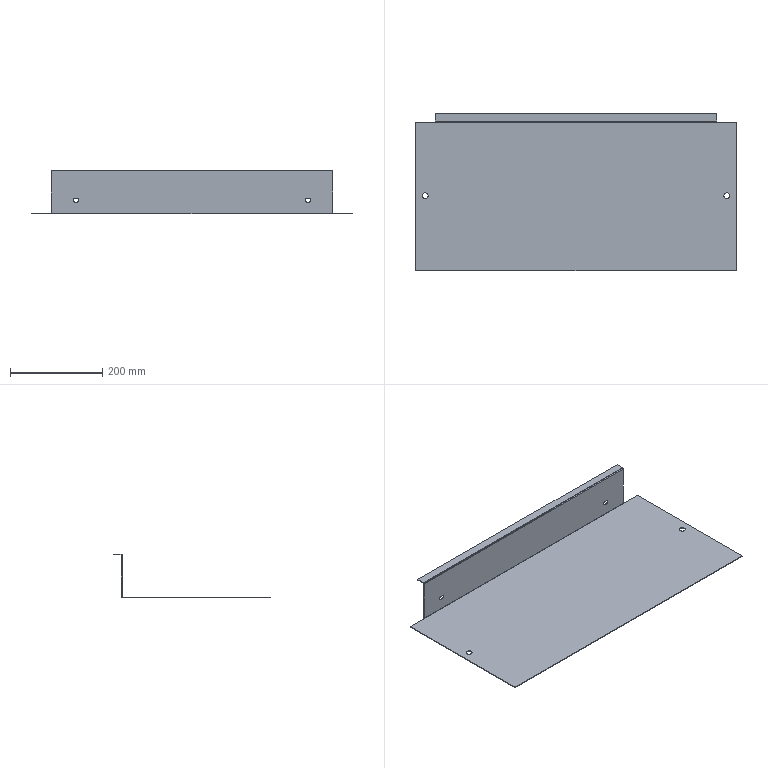Component | SolidWorks | TopCoverPlate-1 | 1 solid | 38 faces | box 697 x 341 x 95 mm | volume 437865 mm3 | plane 26 | cylinder 12 | commonest cylinder face diameters 13 x4 9 x4 4 x2 1 x2
STEP:
#1=COLOUR_RGB('',0.7922,0.8196,0.9333);
#2=FILL_AREA_STYLE_COLOUR('',#1);
#3=FILL_AREA_STYLE('',(#2));
#4=SURFACE_STYLE_FILL_AREA(#3);
#5=SURFACE_SIDE_STYLE('',(#4));
#6=SURFACE_STYLE_USAGE(.BOTH.,#5);
#7=PRESENTATION_STYLE_ASSIGNMENT((#6));
#8=CARTESIAN_POINT('',(-4.863,0.1499,0.05893));
#9=VERTEX_POINT('',#8);
#10=CARTESIAN_POINT('',(-4.863,-0.3619,0.05893));
#11=VERTEX_POINT('',#10);
#12=CARTESIAN_POINT('',(-4.863,-0.106,0.05893));
#13=DIRECTION('',(-0.,-0.,-1.));
#14=DIRECTION('',(-0.,1.,-0.));
#15=AXIS2_PLACEMENT_3D('',#12,#13,#14);
#16=CIRCLE('',#15,0.2559);
#17=EDGE_CURVE('',#9,#11,#16,.T.);
#18=ORIENTED_EDGE('',*,*,#17,.F.);
#19=CARTESIAN_POINT('',(-4.863,0.1499,-0.0001293));
#20=VERTEX_POINT('',#19);
#21=CARTESIAN_POINT('',(-4.863,0.1499,0.05893));
#22=DIRECTION('',(-0.,-0.,-1.));
#23=VECTOR('',#22,39.37);
#24=LINE('',#21,#23);
#25=EDGE_CURVE('',#9,#20,#24,.T.);
#26=ORIENTED_EDGE('',*,*,#25,.T.);
#27=CARTESIAN_POINT('',(-4.863,-0.3619,-0.0001293));
#28=VERTEX_POINT('',#27);
#29=CARTESIAN_POINT('',(-4.863,-0.106,-0.0001293));
#30=DIRECTION('',(-0.,-0.,-1.));
#31=DIRECTION('',(-0.,1.,-0.));
#32=AXIS2_PLACEMENT_3D('',#29,#30,#31);
#33=CIRCLE('',#32,0.2559);
#34=EDGE_CURVE('',#20,#28,#33,.T.);
#35=ORIENTED_EDGE('',*,*,#34,.T.);
#36=CARTESIAN_POINT('',(-4.863,-0.3619,0.05893));
#37=DIRECTION('',(-0.,-0.,-1.));
#38=VECTOR('',#37,39.37);
#39=LINE('',#36,#38);
#40=EDGE_CURVE('',#11,#28,#39,.T.);
#41=ORIENTED_EDGE('',*,*,#40,.F.);
#42=EDGE_LOOP('',(#18,#26,#35,#41));
#43=FACE_OUTER_BOUND('',#42,.T.);
#44=CARTESIAN_POINT('',(-4.863,-0.106,0.05893));
#45=DIRECTION('',(-0.,-0.,-1.));
#46=DIRECTION('',(0.,-1.,0.));
#47=AXIS2_PLACEMENT_3D('',#44,#45,#46);
#48=CYLINDRICAL_SURFACE('',#47,0.2559);
#49=ADVANCED_FACE('',(#43),#48,.F.);
#50=CARTESIAN_POINT('',(20.847,0.1499,0.05893));
#51=VERTEX_POINT('',#50);
#52=CARTESIAN_POINT('',(20.847,-0.3619,0.05893));
#53=VERTEX_POINT('',#52);
#54=CARTESIAN_POINT('',(20.847,-0.106,0.05893));
#55=DIRECTION('',(-0.,-0.,-1.));
#56=DIRECTION('',(0.,-1.,0.));
#57=AXIS2_PLACEMENT_3D('',#54,#55,#56);
#58=CIRCLE('',#57,0.2559);
#59=EDGE_CURVE('',#51,#53,#58,.T.);
#60=ORIENTED_EDGE('',*,*,#59,.F.);
#61=CARTESIAN_POINT('',(20.847,0.1499,-0.0001293));
#62=VERTEX_POINT('',#61);
#63=CARTESIAN_POINT('',(20.847,0.1499,0.05893));
#64=DIRECTION('',(-0.,-0.,-1.));
#65=VECTOR('',#64,39.37);
#66=LINE('',#63,#65);
#67=EDGE_CURVE('',#51,#62,#66,.T.);
#68=ORIENTED_EDGE('',*,*,#67,.T.);
#69=CARTESIAN_POINT('',(20.847,-0.3619,-0.0001293));
#70=VERTEX_POINT('',#69);
#71=CARTESIAN_POINT('',(20.847,-0.106,-0.0001293));
#72=DIRECTION('',(-0.,-0.,-1.));
#73=DIRECTION('',(0.,-1.,0.));
#74=AXIS2_PLACEMENT_3D('',#71,#72,#73);
#75=CIRCLE('',#74,0.2559);
#76=EDGE_CURVE('',#62,#70,#75,.T.);
#77=ORIENTED_EDGE('',*,*,#76,.T.);
#78=CARTESIAN_POINT('',(20.847,-0.3619,0.05893));
#79=DIRECTION('',(-0.,-0.,-1.));
#80=VECTOR('',#79,39.37);
#81=LINE('',#78,#80);
#82=EDGE_CURVE('',#53,#70,#81,.T.);
#83=ORIENTED_EDGE('',*,*,#82,.F.);
#84=EDGE_LOOP('',(#60,#68,#77,#83));
#85=FACE_OUTER_BOUND('',#84,.T.);
#86=CARTESIAN_POINT('',(20.847,-0.106,0.05893));
#87=DIRECTION('',(-0.,-0.,-1.));
#88=DIRECTION('',(0.,-1.,0.));
#89=AXIS2_PLACEMENT_3D('',#86,#87,#88);
#90=CYLINDRICAL_SURFACE('',#89,0.2559);
#91=ADVANCED_FACE('',(#85),#90,.F.);
#92=CARTESIAN_POINT('',(-4.016,6.233,0.07861));
#93=VERTEX_POINT('',#92);
#94=CARTESIAN_POINT('',(20.,6.233,0.07861));
#95=VERTEX_POINT('',#94);
#96=CARTESIAN_POINT('',(-5.729,6.233,0.07861));
#97=DIRECTION('',(1.,0.,-0.));
#98=VECTOR('',#97,39.37);
#99=LINE('',#96,#98);
#100=EDGE_CURVE('',#93,#95,#99,.T.);
#101=ORIENTED_EDGE('',*,*,#100,.T.);
#102=CARTESIAN_POINT('',(20.,6.154,-0.0001293));
#103=VERTEX_POINT('',#102);
#104=CARTESIAN_POINT('',(20.,6.154,0.07861));
#105=DIRECTION('',(-1.,-0.,0.));
#106=DIRECTION('',(0.,-1.,0.));
#107=AXIS2_PLACEMENT_3D('',#104,#105,#106);
#108=CIRCLE('',#107,0.07874);
#109=EDGE_CURVE('',#95,#103,#108,.T.);
#110=ORIENTED_EDGE('',*,*,#109,.T.);
#111=CARTESIAN_POINT('',(-4.016,6.154,-0.0001293));
#112=VERTEX_POINT('',#111);
#113=CARTESIAN_POINT('',(-5.729,6.154,-0.0001293));
#114=DIRECTION('',(1.,0.,-0.));
#115=VECTOR('',#114,39.37);
#116=LINE('',#113,#115);
#117=EDGE_CURVE('',#112,#103,#116,.T.);
#118=ORIENTED_EDGE('',*,*,#117,.F.);
#119=CARTESIAN_POINT('',(-4.016,6.154,0.07861));
#120=DIRECTION('',(1.,0.,-0.));
#121=DIRECTION('',(0.,-1.,0.));
#122=AXIS2_PLACEMENT_3D('',#119,#120,#121);
#123=CIRCLE('',#122,0.07874);
#124=EDGE_CURVE('',#112,#93,#123,.T.);
#125=ORIENTED_EDGE('',*,*,#124,.T.);
#126=EDGE_LOOP('',(#101,#110,#118,#125));
#127=FACE_OUTER_BOUND('',#126,.T.);
#128=CARTESIAN_POINT('',(-5.729,6.154,0.07861));
#129=DIRECTION('',(1.,0.,-0.));
#130=DIRECTION('',(0.,-1.,0.));
#131=AXIS2_PLACEMENT_3D('',#128,#129,#130);
#132=CYLINDRICAL_SURFACE('',#131,0.07874);
#133=ADVANCED_FACE('',(#127),#132,.T.);
#134=CARTESIAN_POINT('',(20.,6.174,0.07861));
#135=VERTEX_POINT('',#134);
#136=CARTESIAN_POINT('',(20.,6.154,0.05893));
#137=VERTEX_POINT('',#136);
#138=CARTESIAN_POINT('',(20.,6.154,0.07861));
#139=DIRECTION('',(-1.,-0.,0.));
#140=DIRECTION('',(0.,-1.,0.));
#141=AXIS2_PLACEMENT_3D('',#138,#139,#140);
#142=CIRCLE('',#141,0.01969);
#143=EDGE_CURVE('',#135,#137,#142,.T.);
#144=ORIENTED_EDGE('',*,*,#143,.F.);
#145=CARTESIAN_POINT('',(-4.016,6.174,0.07861));
#146=VERTEX_POINT('',#145);
#147=CARTESIAN_POINT('',(-5.729,6.174,0.07861));
#148=DIRECTION('',(1.,0.,-0.));
#149=VECTOR('',#148,39.37);
#150=LINE('',#147,#149);
#151=EDGE_CURVE('',#146,#135,#150,.T.);
#152=ORIENTED_EDGE('',*,*,#151,.F.);
#153=CARTESIAN_POINT('',(-4.016,6.154,0.05893));
#154=VERTEX_POINT('',#153);
#155=CARTESIAN_POINT('',(-4.016,6.154,0.07861));
#156=DIRECTION('',(1.,0.,-0.));
#157=DIRECTION('',(0.,1.,0.));
#158=AXIS2_PLACEMENT_3D('',#155,#156,#157);
#159=CIRCLE('',#158,0.01969);
#160=EDGE_CURVE('',#154,#146,#159,.T.);
#161=ORIENTED_EDGE('',*,*,#160,.F.);
#162=CARTESIAN_POINT('',(-5.729,6.154,0.05893));
#163=DIRECTION('',(1.,0.,-0.));
#164=VECTOR('',#163,39.37);
#165=LINE('',#162,#164);
#166=EDGE_CURVE('',#154,#137,#165,.T.);
#167=ORIENTED_EDGE('',*,*,#166,.T.);
#168=EDGE_LOOP('',(#144,#152,#161,#167));
#169=FACE_OUTER_BOUND('',#168,.T.);
#170=CARTESIAN_POINT('',(-5.729,6.154,0.07861));
#171=DIRECTION('',(1.,0.,-0.));
#172=DIRECTION('',(0.,-1.,0.));
#173=AXIS2_PLACEMENT_3D('',#170,#171,#172);
#174=CYLINDRICAL_SURFACE('',#173,0.01969);
#175=ADVANCED_FACE('',(#169),#174,.F.);
#176=CARTESIAN_POINT('',(-4.016,6.252,3.681));
#177=VERTEX_POINT('',#176);
#178=CARTESIAN_POINT('',(20.,6.252,3.681));
#179=VERTEX_POINT('',#178);
#180=CARTESIAN_POINT('',(-5.729,6.252,3.681));
#181=DIRECTION('',(1.,0.,-0.));
#182=VECTOR('',#181,39.37);
#183=LINE('',#180,#182);
#184=EDGE_CURVE('',#177,#179,#183,.T.);
#185=ORIENTED_EDGE('',*,*,#184,.T.);
#186=CARTESIAN_POINT('',(20.,6.233,3.661));
#187=VERTEX_POINT('',#186);
#188=CARTESIAN_POINT('',(20.,6.252,3.661));
#189=DIRECTION('',(-1.,-0.,0.));
#190=DIRECTION('',(0.,-1.,0.));
#191=AXIS2_PLACEMENT_3D('',#188,#189,#190);
#192=CIRCLE('',#191,0.01969);
#193=EDGE_CURVE('',#187,#179,#192,.T.);
#194=ORIENTED_EDGE('',*,*,#193,.F.);
#195=CARTESIAN_POINT('',(-4.016,6.233,3.661));
#196=VERTEX_POINT('',#195);
#197=CARTESIAN_POINT('',(-5.729,6.233,3.661));
#198=DIRECTION('',(1.,0.,-0.));
#199=VECTOR('',#198,39.37);
#200=LINE('',#197,#199);
#201=EDGE_CURVE('',#196,#187,#200,.T.);
#202=ORIENTED_EDGE('',*,*,#201,.F.);
#203=CARTESIAN_POINT('',(-4.016,6.252,3.661));
#204=DIRECTION('',(1.,0.,-0.));
#205=DIRECTION('',(0.,1.,0.));
#206=AXIS2_PLACEMENT_3D('',#203,#204,#205);
#207=CIRCLE('',#206,0.01969);
#208=EDGE_CURVE('',#177,#196,#207,.T.);
#209=ORIENTED_EDGE('',*,*,#208,.F.);
#210=EDGE_LOOP('',(#185,#194,#202,#209));
#211=FACE_OUTER_BOUND('',#210,.T.);
#212=CARTESIAN_POINT('',(-5.729,6.252,3.661));
#213=DIRECTION('',(1.,0.,-0.));
#214=DIRECTION('',(0.,-1.,0.));
#215=AXIS2_PLACEMENT_3D('',#212,#213,#214);
#216=CYLINDRICAL_SURFACE('',#215,0.01969);
#217=ADVANCED_FACE('',(#211),#216,.F.);
#218=CARTESIAN_POINT('',(20.,6.174,3.661));
#219=VERTEX_POINT('',#218);
#220=CARTESIAN_POINT('',(20.,6.252,3.74));
#221=VERTEX_POINT('',#220);
#222=CARTESIAN_POINT('',(20.,6.252,3.661));
#223=DIRECTION('',(-1.,-0.,0.));
#224=DIRECTION('',(0.,-1.,0.));
#225=AXIS2_PLACEMENT_3D('',#222,#223,#224);
#226=CIRCLE('',#225,0.07874);
#227=EDGE_CURVE('',#219,#221,#226,.T.);
#228=ORIENTED_EDGE('',*,*,#227,.T.);
#229=CARTESIAN_POINT('',(-4.016,6.252,3.74));
#230=VERTEX_POINT('',#229);
#231=CARTESIAN_POINT('',(-5.729,6.252,3.74));
#232=DIRECTION('',(1.,0.,-0.));
#233=VECTOR('',#232,39.37);
#234=LINE('',#231,#233);
#235=EDGE_CURVE('',#230,#221,#234,.T.);
#236=ORIENTED_EDGE('',*,*,#235,.F.);
#237=CARTESIAN_POINT('',(-4.016,6.174,3.661));
#238=VERTEX_POINT('',#237);
#239=CARTESIAN_POINT('',(-4.016,6.252,3.661));
#240=DIRECTION('',(1.,0.,-0.));
#241=DIRECTION('',(0.,-1.,0.));
#242=AXIS2_PLACEMENT_3D('',#239,#240,#241);
#243=CIRCLE('',#242,0.07874);
#244=EDGE_CURVE('',#230,#238,#243,.T.);
#245=ORIENTED_EDGE('',*,*,#244,.T.);
#246=CARTESIAN_POINT('',(-5.729,6.174,3.661));
#247=DIRECTION('',(1.,0.,-0.));
#248=VECTOR('',#247,39.37);
#249=LINE('',#246,#248);
#250=EDGE_CURVE('',#238,#219,#249,.T.);
#251=ORIENTED_EDGE('',*,*,#250,.T.);
#252=EDGE_LOOP('',(#228,#236,#245,#251));
#253=FACE_OUTER_BOUND('',#252,.T.);
#254=CARTESIAN_POINT('',(-5.729,6.252,3.661));
#255=DIRECTION('',(1.,0.,-0.));
#256=DIRECTION('',(0.,-1.,0.));
#257=AXIS2_PLACEMENT_3D('',#254,#255,#256);
#258=CYLINDRICAL_SURFACE('',#257,0.07874);
#259=ADVANCED_FACE('',(#253),#258,.T.);
#260=CARTESIAN_POINT('',(17.933,6.233,1.358));
#261=VERTEX_POINT('',#260);
#262=CARTESIAN_POINT('',(17.933,6.233,1.004));
#263=VERTEX_POINT('',#262);
#264=CARTESIAN_POINT('',(17.933,6.233,1.181));
#265=DIRECTION('',(-0.,1.,-0.));
#266=DIRECTION('',(0.,0.,1.));
#267=AXIS2_PLACEMENT_3D('',#264,#265,#266);
#268=CIRCLE('',#267,0.1772);
#269=EDGE_CURVE('',#261,#263,#268,.T.);
#270=ORIENTED_EDGE('',*,*,#269,.F.);
#271=CARTESIAN_POINT('',(17.815,6.233,1.358));
#272=VERTEX_POINT('',#271);
#273=CARTESIAN_POINT('',(17.933,6.233,1.358));
#274=DIRECTION('',(1.,0.,-0.));
#275=VECTOR('',#274,39.37);
#276=LINE('',#273,#275);
#277=EDGE_CURVE('',#272,#261,#276,.T.);
#278=ORIENTED_EDGE('',*,*,#277,.F.);
#279=CARTESIAN_POINT('',(17.815,6.233,1.004));
#280=VERTEX_POINT('',#279);
#281=CARTESIAN_POINT('',(17.815,6.233,1.181));
#282=DIRECTION('',(-0.,1.,-0.));
#283=DIRECTION('',(0.,0.,1.));
#284=AXIS2_PLACEMENT_3D('',#281,#282,#283);
#285=CIRCLE('',#284,0.1772);
#286=EDGE_CURVE('',#280,#272,#285,.T.);
#287=ORIENTED_EDGE('',*,*,#286,.F.);
#288=CARTESIAN_POINT('',(17.933,6.233,1.004));
#289=DIRECTION('',(-1.,-0.,0.));
#290=VECTOR('',#289,39.37);
#291=LINE('',#288,#290);
#292=EDGE_CURVE('',#263,#280,#291,.T.);
#293=ORIENTED_EDGE('',*,*,#292,.F.);
#294=EDGE_LOOP('',(#270,#278,#287,#293));
#295=FACE_BOUND('',#294,.T.);
#296=CARTESIAN_POINT('',(-1.949,6.233,1.004));
#297=VERTEX_POINT('',#296);
#298=CARTESIAN_POINT('',(-1.949,6.233,1.358));
#299=VERTEX_POINT('',#298);
#300=CARTESIAN_POINT('',(-1.949,6.233,1.181));
#301=DIRECTION('',(-0.,1.,-0.));
#302=DIRECTION('',(-0.,0.,-1.));
#303=AXIS2_PLACEMENT_3D('',#300,#301,#302);
#304=CIRCLE('',#303,0.1772);
#305=EDGE_CURVE('',#297,#299,#304,.T.);
#306=ORIENTED_EDGE('',*,*,#305,.F.);
#307=CARTESIAN_POINT('',(-1.831,6.233,1.004));
#308=VERTEX_POINT('',#307);
#309=CARTESIAN_POINT('',(-1.949,6.233,1.004));
#310=DIRECTION('',(-1.,-0.,0.));
#311=VECTOR('',#310,39.37);
#312=LINE('',#309,#311);
#313=EDGE_CURVE('',#308,#297,#312,.T.);
#314=ORIENTED_EDGE('',*,*,#313,.F.);
#315=CARTESIAN_POINT('',(-1.831,6.233,1.358));
#316=VERTEX_POINT('',#315);
#317=CARTESIAN_POINT('',(-1.831,6.233,1.181));
#318=DIRECTION('',(-0.,1.,-0.));
#319=DIRECTION('',(-0.,0.,-1.));
#320=AXIS2_PLACEMENT_3D('',#317,#318,#319);
#321=CIRCLE('',#320,0.1772);
#322=EDGE_CURVE('',#316,#308,#321,.T.);
#323=ORIENTED_EDGE('',*,*,#322,.F.);
#324=CARTESIAN_POINT('',(-1.949,6.233,1.358));
#325=DIRECTION('',(1.,0.,-0.));
#326=VECTOR('',#325,39.37);
#327=LINE('',#324,#326);
#328=EDGE_CURVE('',#299,#316,#327,.T.);
#329=ORIENTED_EDGE('',*,*,#328,.F.);
#330=EDGE_LOOP('',(#306,#314,#323,#329));
#331=FACE_BOUND('',#330,.T.);
#332=ORIENTED_EDGE('',*,*,#201,.T.);
#333=CARTESIAN_POINT('',(20.,6.233,-0.0001293));
#334=DIRECTION('',(-0.,-0.,-1.));
#335=VECTOR('',#334,39.37);
#336=LINE('',#333,#335);
#337=EDGE_CURVE('',#187,#95,#336,.T.);
#338=ORIENTED_EDGE('',*,*,#337,.T.);
#339=ORIENTED_EDGE('',*,*,#100,.F.);
#340=CARTESIAN_POINT('',(-4.016,6.233,0.07861));
#341=DIRECTION('',(-0.,-0.,-1.));
#342=VECTOR('',#341,39.37);
#343=LINE('',#340,#342);
#344=EDGE_CURVE('',#196,#93,#343,.T.);
#345=ORIENTED_EDGE('',*,*,#344,.F.);
#346=EDGE_LOOP('',(#332,#338,#339,#345));
#347=FACE_OUTER_BOUND('',#346,.T.);
#348=CARTESIAN_POINT('',(-5.729,6.233,-0.0001293));
#349=DIRECTION('',(-0.,1.,-0.));
#350=DIRECTION('',(-0.,-0.,-1.));
#351=AXIS2_PLACEMENT_3D('',#348,#349,#350);
#352=PLANE('',#351);
#353=ADVANCED_FACE('',(#295,#331,#347),#352,.T.);
#354=CARTESIAN_POINT('',(17.815,6.174,1.358));
#355=VERTEX_POINT('',#354);
#356=CARTESIAN_POINT('',(17.933,6.174,1.358));
#357=VERTEX_POINT('',#356);
#358=CARTESIAN_POINT('',(17.933,6.174,1.358));
#359=DIRECTION('',(1.,0.,-0.));
#360=VECTOR('',#359,39.37);
#361=LINE('',#358,#360);
#362=EDGE_CURVE('',#355,#357,#361,.T.);
#363=ORIENTED_EDGE('',*,*,#362,.T.);
#364=CARTESIAN_POINT('',(17.933,6.174,1.004));
#365=VERTEX_POINT('',#364);
#366=CARTESIAN_POINT('',(17.933,6.174,1.181));
#367=DIRECTION('',(-0.,1.,-0.));
#368=DIRECTION('',(0.,0.,1.));
#369=AXIS2_PLACEMENT_3D('',#366,#367,#368);
#370=CIRCLE('',#369,0.1772);
#371=EDGE_CURVE('',#357,#365,#370,.T.);
#372=ORIENTED_EDGE('',*,*,#371,.T.);
#373=CARTESIAN_POINT('',(17.815,6.174,1.004));
#374=VERTEX_POINT('',#373);
#375=CARTESIAN_POINT('',(17.933,6.174,1.004));
#376=DIRECTION('',(-1.,-0.,0.));
#377=VECTOR('',#376,39.37);
#378=LINE('',#375,#377);
#379=EDGE_CURVE('',#365,#374,#378,.T.);
#380=ORIENTED_EDGE('',*,*,#379,.T.);
#381=CARTESIAN_POINT('',(17.815,6.174,1.181));
#382=DIRECTION('',(-0.,1.,-0.));
#383=DIRECTION('',(0.,0.,1.));
#384=AXIS2_PLACEMENT_3D('',#381,#382,#383);
#385=CIRCLE('',#384,0.1772);
#386=EDGE_CURVE('',#374,#355,#385,.T.);
#387=ORIENTED_EDGE('',*,*,#386,.T.);
#388=EDGE_LOOP('',(#363,#372,#380,#387));
#389=FACE_BOUND('',#388,.T.);
#390=CARTESIAN_POINT('',(-1.831,6.174,1.004));
#391=VERTEX_POINT('',#390);
#392=CARTESIAN_POINT('',(-1.949,6.174,1.004));
#393=VERTEX_POINT('',#392);
#394=CARTESIAN_POINT('',(-1.949,6.174,1.004));
#395=DIRECTION('',(-1.,-0.,0.));
#396=VECTOR('',#395,39.37);
#397=LINE('',#394,#396);
#398=EDGE_CURVE('',#391,#393,#397,.T.);
#399=ORIENTED_EDGE('',*,*,#398,.T.);
#400=CARTESIAN_POINT('',(-1.949,6.174,1.358));
#401=VERTEX_POINT('',#400);
#402=CARTESIAN_POINT('',(-1.949,6.174,1.181));
#403=DIRECTION('',(-0.,1.,-0.));
#404=DIRECTION('',(-0.,0.,-1.));
#405=AXIS2_PLACEMENT_3D('',#402,#403,#404);
#406=CIRCLE('',#405,0.1772);
#407=EDGE_CURVE('',#393,#401,#406,.T.);
#408=ORIENTED_EDGE('',*,*,#407,.T.);
#409=CARTESIAN_POINT('',(-1.831,6.174,1.358));
#410=VERTEX_POINT('',#409);
#411=CARTESIAN_POINT('',(-1.949,6.174,1.358));
#412=DIRECTION('',(1.,0.,-0.));
#413=VECTOR('',#412,39.37);
#414=LINE('',#411,#413);
#415=EDGE_CURVE('',#401,#410,#414,.T.);
#416=ORIENTED_EDGE('',*,*,#415,.T.);
#417=CARTESIAN_POINT('',(-1.831,6.174,1.181));
#418=DIRECTION('',(-0.,1.,-0.));
#419=DIRECTION('',(-0.,0.,-1.));
#420=AXIS2_PLACEMENT_3D('',#417,#418,#419);
#421=CIRCLE('',#420,0.1772);
#422=EDGE_CURVE('',#410,#391,#421,.T.);
#423=ORIENTED_EDGE('',*,*,#422,.T.);
#424=EDGE_LOOP('',(#399,#408,#416,#423));
#425=FACE_BOUND('',#424,.T.);
#426=CARTESIAN_POINT('',(20.,6.174,0.07861));
#427=DIRECTION('',(-0.,-0.,-1.));
#428=VECTOR('',#427,39.37);
#429=LINE('',#426,#428);
#430=EDGE_CURVE('',#219,#135,#429,.T.);
#431=ORIENTED_EDGE('',*,*,#430,.F.);
#432=ORIENTED_EDGE('',*,*,#250,.F.);
#433=CARTESIAN_POINT('',(-4.016,6.174,-0.0001293));
#434=DIRECTION('',(-0.,-0.,-1.));
#435=VECTOR('',#434,39.37);
#436=LINE('',#433,#435);
#437=EDGE_CURVE('',#238,#146,#436,.T.);
#438=ORIENTED_EDGE('',*,*,#437,.T.);
#439=ORIENTED_EDGE('',*,*,#151,.T.);
#440=EDGE_LOOP('',(#431,#432,#438,#439));
#441=FACE_OUTER_BOUND('',#440,.T.);
#442=CARTESIAN_POINT('',(-5.729,6.174,-0.0001293));
#443=DIRECTION('',(-0.,1.,-0.));
#444=DIRECTION('',(-0.,-0.,-1.));
#445=AXIS2_PLACEMENT_3D('',#442,#443,#444);
#446=PLANE('',#445);
#447=ADVANCED_FACE('',(#389,#425,#441),#446,.F.);
#448=CARTESIAN_POINT('',(20.,6.922,3.74));
#449=VERTEX_POINT('',#448);
#450=CARTESIAN_POINT('',(20.,6.922,3.74));
#451=DIRECTION('',(0.,-1.,0.));
#452=VECTOR('',#451,39.37);
#453=LINE('',#450,#452);
#454=EDGE_CURVE('',#449,#221,#453,.T.);
#455=ORIENTED_EDGE('',*,*,#454,.F.);
#456=CARTESIAN_POINT('',(-4.016,6.922,3.74));
#457=VERTEX_POINT('',#456);
#458=CARTESIAN_POINT('',(-5.729,6.922,3.74));
#459=DIRECTION('',(1.,0.,-0.));
#460=VECTOR('',#459,39.37);
#461=LINE('',#458,#460);
#462=EDGE_CURVE('',#457,#449,#461,.T.);
#463=ORIENTED_EDGE('',*,*,#462,.F.);
#464=CARTESIAN_POINT('',(-4.016,6.233,3.74));
#465=DIRECTION('',(0.,-1.,0.));
#466=VECTOR('',#465,39.37);
#467=LINE('',#464,#466);
#468=EDGE_CURVE('',#457,#230,#467,.T.);
#469=ORIENTED_EDGE('',*,*,#468,.T.);
#470=ORIENTED_EDGE('',*,*,#235,.T.);
#471=EDGE_LOOP('',(#455,#463,#469,#470));
#472=FACE_OUTER_BOUND('',#471,.T.);
#473=CARTESIAN_POINT('',(-5.729,6.233,3.74));
#474=DIRECTION('',(-0.,-0.,-1.));
#475=DIRECTION('',(-1.,-0.,0.));
#476=AXIS2_PLACEMENT_3D('',#473,#474,#475);
#477=PLANE('',#476);
#478=ADVANCED_FACE('',(#472),#477,.F.);
#479=ORIENTED_EDGE('',*,*,#462,.T.);
#480=CARTESIAN_POINT('',(20.,6.922,3.681));
#481=VERTEX_POINT('',#480);
#482=CARTESIAN_POINT('',(20.,6.922,3.74));
#483=DIRECTION('',(-0.,-0.,-1.));
#484=VECTOR('',#483,39.37);
#485=LINE('',#482,#484);
#486=EDGE_CURVE('',#449,#481,#485,.T.);
#487=ORIENTED_EDGE('',*,*,#486,.T.);
#488=CARTESIAN_POINT('',(-4.016,6.922,3.681));
#489=VERTEX_POINT('',#488);
#490=CARTESIAN_POINT('',(-5.729,6.922,3.681));
#491=DIRECTION('',(1.,0.,-0.));
#492=VECTOR('',#491,39.37);
#493=LINE('',#490,#492);
#494=EDGE_CURVE('',#489,#481,#493,.T.);
#495=ORIENTED_EDGE('',*,*,#494,.F.);
#496=CARTESIAN_POINT('',(-4.016,6.922,3.681));
#497=DIRECTION('',(0.,0.,1.));
#498=VECTOR('',#497,39.37);
#499=LINE('',#496,#498);
#500=EDGE_CURVE('',#489,#457,#499,.T.);
#501=ORIENTED_EDGE('',*,*,#500,.T.);
#502=EDGE_LOOP('',(#479,#487,#495,#501));
#503=FACE_OUTER_BOUND('',#502,.T.);
#504=CARTESIAN_POINT('',(-5.729,6.922,3.681));
#505=DIRECTION('',(-0.,1.,0.));
#506=DIRECTION('',(1.,0.,-0.));
#507=AXIS2_PLACEMENT_3D('',#504,#505,#506);
#508=PLANE('',#507);
#509=ADVANCED_FACE('',(#503),#508,.T.);
#510=ORIENTED_EDGE('',*,*,#494,.T.);
#511=CARTESIAN_POINT('',(20.,6.233,3.681));
#512=DIRECTION('',(0.,-1.,0.));
#513=VECTOR('',#512,39.37);
#514=LINE('',#511,#513);
#515=EDGE_CURVE('',#481,#179,#514,.T.);
#516=ORIENTED_EDGE('',*,*,#515,.T.);
#517=ORIENTED_EDGE('',*,*,#184,.F.);
#518=CARTESIAN_POINT('',(-4.016,6.252,3.681));
#519=DIRECTION('',(0.,-1.,0.));
#520=VECTOR('',#519,39.37);
#521=LINE('',#518,#520);
#522=EDGE_CURVE('',#489,#177,#521,.T.);
#523=ORIENTED_EDGE('',*,*,#522,.F.);
#524=EDGE_LOOP('',(#510,#516,#517,#523));
#525=FACE_OUTER_BOUND('',#524,.T.);
#526=CARTESIAN_POINT('',(-5.729,6.233,3.681));
#527=DIRECTION('',(-0.,-0.,-1.));
#528=DIRECTION('',(-1.,-0.,0.));
#529=AXIS2_PLACEMENT_3D('',#526,#527,#528);
#530=PLANE('',#529);
#531=ADVANCED_FACE('',(#525),#530,.T.);
#532=CARTESIAN_POINT('',(21.712,-6.425,0.05893));
#533=VERTEX_POINT('',#532);
#534=CARTESIAN_POINT('',(21.712,6.154,0.05893));
#535=VERTEX_POINT('',#534);
#536=CARTESIAN_POINT('',(21.712,6.233,0.05893));
#537=DIRECTION('',(-0.,1.,-0.));
#538=VECTOR('',#537,39.37);
#539=LINE('',#536,#538);
#540=EDGE_CURVE('',#533,#535,#539,.T.);
#541=ORIENTED_EDGE('',*,*,#540,.F.);
#542=CARTESIAN_POINT('',(21.712,-6.425,-0.0001293));
#543=VERTEX_POINT('',#542);
#544=CARTESIAN_POINT('',(21.712,-6.425,0.07861));
#545=DIRECTION('',(-0.,-0.,-1.));
#546=VECTOR('',#545,39.37);
#547=LINE('',#544,#546);
#548=EDGE_CURVE('',#533,#543,#547,.T.);
#549=ORIENTED_EDGE('',*,*,#548,.T.);
#550=CARTESIAN_POINT('',(21.712,6.154,-0.0001293));
#551=VERTEX_POINT('',#550);
#552=CARTESIAN_POINT('',(21.712,6.233,-0.0001293));
#553=DIRECTION('',(-0.,1.,-0.));
#554=VECTOR('',#553,39.37);
#555=LINE('',#552,#554);
#556=EDGE_CURVE('',#543,#551,#555,.T.);
#557=ORIENTED_EDGE('',*,*,#556,.T.);
#558=CARTESIAN_POINT('',(21.712,6.154,-0.0001293));
#559=DIRECTION('',(0.,0.,1.));
#560=VECTOR('',#559,39.37);
#561=LINE('',#558,#560);
#562=EDGE_CURVE('',#551,#535,#561,.T.);
#563=ORIENTED_EDGE('',*,*,#562,.T.);
#564=EDGE_LOOP('',(#541,#549,#557,#563));
#565=FACE_OUTER_BOUND('',#564,.T.);
#566=CARTESIAN_POINT('',(21.712,6.174,0.07861));
#567=DIRECTION('',(1.,0.,-0.));
#568=DIRECTION('',(0.,-1.,0.));
#569=AXIS2_PLACEMENT_3D('',#566,#567,#568);
#570=PLANE('',#569);
#571=ADVANCED_FACE('',(#565),#570,.T.);
#572=CARTESIAN_POINT('',(-4.863,-0.106,-0.0001293));
#573=DIRECTION('',(-0.,-0.,-1.));
#574=DIRECTION('',(-0.,1.,-0.));
#575=AXIS2_PLACEMENT_3D('',#572,#573,#574);
#576=CIRCLE('',#575,0.2559);
#577=EDGE_CURVE('',#28,#20,#576,.T.);
#578=ORIENTED_EDGE('',*,*,#577,.F.);
#579=ORIENTED_EDGE('',*,*,#34,.F.);
#580=EDGE_LOOP('',(#578,#579));
#581=FACE_BOUND('',#580,.T.);
#582=CARTESIAN_POINT('',(20.847,-0.106,-0.0001293));
#583=DIRECTION('',(-0.,-0.,-1.));
#584=DIRECTION('',(0.,-1.,0.));
#585=AXIS2_PLACEMENT_3D('',#582,#583,#584);
#586=CIRCLE('',#585,0.2559);
#587=EDGE_CURVE('',#70,#62,#586,.T.);
#588=ORIENTED_EDGE('',*,*,#587,.F.);
#589=ORIENTED_EDGE('',*,*,#76,.F.);
#590=EDGE_LOOP('',(#588,#589));
#591=FACE_BOUND('',#590,.T.);
#592=CARTESIAN_POINT('',(-5.65,-6.504,-0.0001293));
#593=VERTEX_POINT('',#592);
#594=CARTESIAN_POINT('',(21.634,-6.504,-0.0001293));
#595=VERTEX_POINT('',#594);
#596=CARTESIAN_POINT('',(-5.729,-6.504,-0.0001293));
#597=DIRECTION('',(1.,0.,-0.));
#598=VECTOR('',#597,39.37);
#599=LINE('',#596,#598);
#600=EDGE_CURVE('',#593,#595,#599,.T.);
#601=ORIENTED_EDGE('',*,*,#600,.F.);
#602=CARTESIAN_POINT('',(-5.729,-6.425,-0.0001293));
#603=VERTEX_POINT('',#602);
#604=CARTESIAN_POINT('',(-12.057,-0.09617,-0.0001293));
#605=DIRECTION('',(-0.7071,0.7071,0.));
#606=VECTOR('',#605,39.37);
#607=LINE('',#604,#606);
#608=EDGE_CURVE('',#593,#603,#607,.T.);
#609=ORIENTED_EDGE('',*,*,#608,.T.);
#610=CARTESIAN_POINT('',(-5.729,6.154,-0.0001293));
#611=VERTEX_POINT('',#610);
#612=CARTESIAN_POINT('',(-5.729,6.233,-0.0001293));
#613=DIRECTION('',(-0.,1.,-0.));
#614=VECTOR('',#613,39.37);
#615=LINE('',#612,#614);
#616=EDGE_CURVE('',#603,#611,#615,.T.);
#617=ORIENTED_EDGE('',*,*,#616,.T.);
#618=CARTESIAN_POINT('',(-5.729,6.154,-0.0001293));
#619=DIRECTION('',(1.,0.,-0.));
#620=VECTOR('',#619,39.37);
#621=LINE('',#618,#620);
#622=EDGE_CURVE('',#611,#112,#621,.T.);
#623=ORIENTED_EDGE('',*,*,#622,.T.);
#624=ORIENTED_EDGE('',*,*,#117,.T.);
#625=CARTESIAN_POINT('',(-5.729,6.154,-0.0001293));
#626=DIRECTION('',(1.,0.,-0.));
#627=VECTOR('',#626,39.37);
#628=LINE('',#625,#627);
#629=EDGE_CURVE('',#103,#551,#628,.T.);
#630=ORIENTED_EDGE('',*,*,#629,.T.);
#631=ORIENTED_EDGE('',*,*,#556,.F.);
#632=CARTESIAN_POINT('',(14.321,-13.817,-0.0001293));
#633=DIRECTION('',(-0.7071,-0.7071,0.));
#634=VECTOR('',#633,39.37);
#635=LINE('',#632,#634);
#636=EDGE_CURVE('',#543,#595,#635,.T.);
#637=ORIENTED_EDGE('',*,*,#636,.T.);
#638=EDGE_LOOP('',(#601,#609,#617,#623,#624,#630,#631,#637));
#639=FACE_OUTER_BOUND('',#638,.T.);
#640=CARTESIAN_POINT('',(-5.729,6.233,-0.0001293));
#641=DIRECTION('',(-0.,-0.,-1.));
#642=DIRECTION('',(0.,-1.,0.));
#643=AXIS2_PLACEMENT_3D('',#640,#641,#642);
#644=PLANE('',#643);
#645=ADVANCED_FACE('',(#581,#591,#639),#644,.T.);
#646=CARTESIAN_POINT('',(-5.65,-6.504,0.05893));
#647=VERTEX_POINT('',#646);
#648=CARTESIAN_POINT('',(21.634,-6.504,0.05893));
#649=VERTEX_POINT('',#648);
#650=CARTESIAN_POINT('',(-5.729,-6.504,0.05893));
#651=DIRECTION('',(1.,0.,-0.));
#652=VECTOR('',#651,39.37);
#653=LINE('',#650,#652);
#654=EDGE_CURVE('',#647,#649,#653,.T.);
#655=ORIENTED_EDGE('',*,*,#654,.F.);
#656=CARTESIAN_POINT('',(-5.65,-6.504,-0.0001293));
#657=DIRECTION('',(-0.,-0.,-1.));
#658=VECTOR('',#657,39.37);
#659=LINE('',#656,#658);
#660=EDGE_CURVE('',#647,#593,#659,.T.);
#661=ORIENTED_EDGE('',*,*,#660,.T.);
#662=ORIENTED_EDGE('',*,*,#600,.T.);
#663=CARTESIAN_POINT('',(21.634,-6.504,0.05893));
#664=DIRECTION('',(0.,0.,1.));
#665=VECTOR('',#664,39.37);
#666=LINE('',#663,#665);
#667=EDGE_CURVE('',#595,#649,#666,.T.);
#668=ORIENTED_EDGE('',*,*,#667,.T.);
#669=EDGE_LOOP('',(#655,#661,#662,#668));
#670=FACE_OUTER_BOUND('',#669,.T.);
#671=CARTESIAN_POINT('',(-5.729,-6.504,0.05893));
#672=DIRECTION('',(0.,-1.,0.));
#673=DIRECTION('',(-1.,-0.,0.));
#674=AXIS2_PLACEMENT_3D('',#671,#672,#673);
#675=PLANE('',#674);
#676=ADVANCED_FACE('',(#670),#675,.T.);
#677=CARTESIAN_POINT('',(-4.863,-0.106,0.05893));
#678=DIRECTION('',(-0.,-0.,-1.));
#679=DIRECTION('',(-0.,1.,-0.));
#680=AXIS2_PLACEMENT_3D('',#677,#678,#679);
#681=CIRCLE('',#680,0.2559);
#682=EDGE_CURVE('',#11,#9,#681,.T.);
#683=ORIENTED_EDGE('',*,*,#682,.T.);
#684=ORIENTED_EDGE('',*,*,#17,.T.);
#685=EDGE_LOOP('',(#683,#684));
#686=FACE_BOUND('',#685,.T.);
#687=CARTESIAN_POINT('',(20.847,-0.106,0.05893));
#688=DIRECTION('',(-0.,-0.,-1.));
#689=DIRECTION('',(0.,-1.,0.));
#690=AXIS2_PLACEMENT_3D('',#687,#688,#689);
#691=CIRCLE('',#690,0.2559);
#692=EDGE_CURVE('',#53,#51,#691,.T.);
#693=ORIENTED_EDGE('',*,*,#692,.T.);
#694=ORIENTED_EDGE('',*,*,#59,.T.);
#695=EDGE_LOOP('',(#693,#694));
#696=FACE_BOUND('',#695,.T.);
#697=CARTESIAN_POINT('',(-5.729,-6.425,0.05893));
#698=VERTEX_POINT('',#697);
#699=CARTESIAN_POINT('',(-5.729,6.154,0.05893));
#700=VERTEX_POINT('',#699);
#701=CARTESIAN_POINT('',(-5.729,6.233,0.05893));
#702=DIRECTION('',(-0.,1.,-0.));
#703=VECTOR('',#702,39.37);
#704=LINE('',#701,#703);
#705=EDGE_CURVE('',#698,#700,#704,.T.);
#706=ORIENTED_EDGE('',*,*,#705,.F.);
#707=CARTESIAN_POINT('',(-5.65,-6.504,0.05893));
#708=DIRECTION('',(0.7071,-0.7071,-0.));
#709=VECTOR('',#708,39.37);
#710=LINE('',#707,#709);
#711=EDGE_CURVE('',#698,#647,#710,.T.);
#712=ORIENTED_EDGE('',*,*,#711,.T.);
#713=ORIENTED_EDGE('',*,*,#654,.T.);
#714=CARTESIAN_POINT('',(21.712,-6.425,0.05893));
#715=DIRECTION('',(0.7071,0.7071,-0.));
#716=VECTOR('',#715,39.37);
#717=LINE('',#714,#716);
#718=EDGE_CURVE('',#649,#533,#717,.T.);
#719=ORIENTED_EDGE('',*,*,#718,.T.);
#720=ORIENTED_EDGE('',*,*,#540,.T.);
#721=CARTESIAN_POINT('',(20.,6.154,0.05893));
#722=DIRECTION('',(1.,0.,-0.));
#723=VECTOR('',#722,39.37);
#724=LINE('',#721,#723);
#725=EDGE_CURVE('',#137,#535,#724,.T.);
#726=ORIENTED_EDGE('',*,*,#725,.F.);
#727=ORIENTED_EDGE('',*,*,#166,.F.);
#728=CARTESIAN_POINT('',(-5.729,6.154,0.05893));
#729=DIRECTION('',(1.,0.,-0.));
#730=VECTOR('',#729,39.37);
#731=LINE('',#728,#730);
#732=EDGE_CURVE('',#700,#154,#731,.T.);
#733=ORIENTED_EDGE('',*,*,#732,.F.);
#734=EDGE_LOOP('',(#706,#712,#713,#719,#720,#726,#727,#733));
#735=FACE_OUTER_BOUND('',#734,.T.);
#736=CARTESIAN_POINT('',(-5.729,6.233,0.05893));
#737=DIRECTION('',(-0.,-0.,-1.));
#738=DIRECTION('',(0.,-1.,0.));
#739=AXIS2_PLACEMENT_3D('',#736,#737,#738);
#740=PLANE('',#739);
#741=ADVANCED_FACE('',(#686,#696,#735),#740,.F.);
#742=ORIENTED_EDGE('',*,*,#616,.F.);
#743=CARTESIAN_POINT('',(-5.729,-6.425,0.05893));
#744=DIRECTION('',(0.,0.,1.));
#745=VECTOR('',#744,39.37);
#746=LINE('',#743,#745);
#747=EDGE_CURVE('',#603,#698,#746,.T.);
#748=ORIENTED_EDGE('',*,*,#747,.T.);
#749=ORIENTED_EDGE('',*,*,#705,.T.);
#750=CARTESIAN_POINT('',(-5.729,6.154,0.05893));
#751=DIRECTION('',(-0.,-0.,-1.));
#752=VECTOR('',#751,39.37);
#753=LINE('',#750,#752);
#754=EDGE_CURVE('',#700,#611,#753,.T.);
#755=ORIENTED_EDGE('',*,*,#754,.T.);
#756=EDGE_LOOP('',(#742,#748,#749,#755));
#757=FACE_OUTER_BOUND('',#756,.T.);
#758=CARTESIAN_POINT('',(-5.729,6.252,3.661));
#759=DIRECTION('',(1.,0.,-0.));
#760=DIRECTION('',(0.,-1.,0.));
#761=AXIS2_PLACEMENT_3D('',#758,#759,#760);
#762=PLANE('',#761);
#763=ADVANCED_FACE('',(#757),#762,.F.);
#764=ORIENTED_EDGE('',*,*,#711,.F.);
#765=ORIENTED_EDGE('',*,*,#747,.F.);
#766=ORIENTED_EDGE('',*,*,#608,.F.);
#767=ORIENTED_EDGE('',*,*,#660,.F.);
#768=EDGE_LOOP('',(#764,#765,#766,#767));
#769=FACE_OUTER_BOUND('',#768,.T.);
#770=CARTESIAN_POINT('',(-5.65,-6.504,0.05893));
#771=DIRECTION('',(-0.7071,-0.7071,0.));
#772=DIRECTION('',(0.,0.,1.));
#773=AXIS2_PLACEMENT_3D('',#770,#771,#772);
#774=PLANE('',#773);
#775=ADVANCED_FACE('',(#769),#774,.T.);
#776=ORIENTED_EDGE('',*,*,#718,.F.);
#777=ORIENTED_EDGE('',*,*,#667,.F.);
#778=ORIENTED_EDGE('',*,*,#636,.F.);
#779=ORIENTED_EDGE('',*,*,#548,.F.);
#780=EDGE_LOOP('',(#776,#777,#778,#779));
#781=FACE_OUTER_BOUND('',#780,.T.);
#782=CARTESIAN_POINT('',(21.712,-6.425,0.07861));
#783=DIRECTION('',(-0.7071,0.7071,0.));
#784=DIRECTION('',(-0.,-0.,-1.));
#785=AXIS2_PLACEMENT_3D('',#782,#783,#784);
#786=PLANE('',#785);
#787=ADVANCED_FACE('',(#781),#786,.F.);
#788=ORIENTED_EDGE('',*,*,#67,.F.);
#789=ORIENTED_EDGE('',*,*,#692,.F.);
#790=ORIENTED_EDGE('',*,*,#82,.T.);
#791=ORIENTED_EDGE('',*,*,#587,.T.);
#792=EDGE_LOOP('',(#788,#789,#790,#791));
#793=FACE_OUTER_BOUND('',#792,.T.);
#794=CARTESIAN_POINT('',(20.847,-0.106,0.05893));
#795=DIRECTION('',(-0.,-0.,-1.));
#796=DIRECTION('',(0.,-1.,0.));
#797=AXIS2_PLACEMENT_3D('',#794,#795,#796);
#798=CYLINDRICAL_SURFACE('',#797,0.2559);
#799=ADVANCED_FACE('',(#793),#798,.F.);
#800=ORIENTED_EDGE('',*,*,#25,.F.);
#801=ORIENTED_EDGE('',*,*,#682,.F.);
#802=ORIENTED_EDGE('',*,*,#40,.T.);
#803=ORIENTED_EDGE('',*,*,#577,.T.);
#804=EDGE_LOOP('',(#800,#801,#802,#803));
#805=FACE_OUTER_BOUND('',#804,.T.);
#806=CARTESIAN_POINT('',(-4.863,-0.106,0.05893));
#807=DIRECTION('',(-0.,-0.,-1.));
#808=DIRECTION('',(0.,-1.,0.));
#809=AXIS2_PLACEMENT_3D('',#806,#807,#808);
#810=CYLINDRICAL_SURFACE('',#809,0.2559);
#811=ADVANCED_FACE('',(#805),#810,.F.);
#812=ORIENTED_EDGE('',*,*,#500,.F.);
#813=ORIENTED_EDGE('',*,*,#522,.T.);
#814=CARTESIAN_POINT('',(-4.016,6.252,3.681));
#815=DIRECTION('',(0.,0.,1.));
#816=VECTOR('',#815,39.37);
#817=LINE('',#814,#816);
#818=EDGE_CURVE('',#177,#230,#817,.T.);
#819=ORIENTED_EDGE('',*,*,#818,.T.);
#820=ORIENTED_EDGE('',*,*,#468,.F.);
#821=EDGE_LOOP('',(#812,#813,#819,#820));
#822=FACE_OUTER_BOUND('',#821,.T.);
#823=CARTESIAN_POINT('',(-4.016,6.252,3.681));
#824=DIRECTION('',(1.,0.,-0.));
#825=DIRECTION('',(0.,-1.,0.));
#826=AXIS2_PLACEMENT_3D('',#823,#824,#825);
#827=PLANE('',#826);
#828=ADVANCED_FACE('',(#822),#827,.F.);
#829=CARTESIAN_POINT('',(-4.016,6.233,3.661));
#830=DIRECTION('',(0.,-1.,0.));
#831=VECTOR('',#830,39.37);
#832=LINE('',#829,#831);
#833=EDGE_CURVE('',#196,#238,#832,.T.);
#834=ORIENTED_EDGE('',*,*,#833,.F.);
#835=ORIENTED_EDGE('',*,*,#344,.T.);
#836=CARTESIAN_POINT('',(-4.016,6.233,0.07861));
#837=DIRECTION('',(0.,-1.,0.));
#838=VECTOR('',#837,39.37);
#839=LINE('',#836,#838);
#840=EDGE_CURVE('',#93,#146,#839,.T.);
#841=ORIENTED_EDGE('',*,*,#840,.T.);
#842=ORIENTED_EDGE('',*,*,#437,.F.);
#843=EDGE_LOOP('',(#834,#835,#841,#842));
#844=FACE_OUTER_BOUND('',#843,.T.);
#845=CARTESIAN_POINT('',(-4.016,6.233,0.07861));
#846=DIRECTION('',(1.,0.,-0.));
#847=DIRECTION('',(-0.,-0.,-1.));
#848=AXIS2_PLACEMENT_3D('',#845,#846,#847);
#849=PLANE('',#848);
#850=ADVANCED_FACE('',(#844),#849,.F.);
#851=ORIENTED_EDGE('',*,*,#754,.F.);
#852=ORIENTED_EDGE('',*,*,#732,.T.);
#853=CARTESIAN_POINT('',(-4.016,6.154,0.05893));
#854=DIRECTION('',(-0.,-0.,-1.));
#855=VECTOR('',#854,39.37);
#856=LINE('',#853,#855);
#857=EDGE_CURVE('',#154,#112,#856,.T.);
#858=ORIENTED_EDGE('',*,*,#857,.T.);
#859=ORIENTED_EDGE('',*,*,#622,.F.);
#860=EDGE_LOOP('',(#851,#852,#858,#859));
#861=FACE_OUTER_BOUND('',#860,.T.);
#862=CARTESIAN_POINT('',(-4.872,6.154,0.05893));
#863=DIRECTION('',(-0.,1.,0.));
#864=DIRECTION('',(1.,0.,-0.));
#865=AXIS2_PLACEMENT_3D('',#862,#863,#864);
#866=PLANE('',#865);
#867=ADVANCED_FACE('',(#861),#866,.T.);
#868=ORIENTED_EDGE('',*,*,#160,.T.);
#869=ORIENTED_EDGE('',*,*,#840,.F.);
#870=ORIENTED_EDGE('',*,*,#124,.F.);
#871=ORIENTED_EDGE('',*,*,#857,.F.);
#872=EDGE_LOOP('',(#868,#869,#870,#871));
#873=FACE_OUTER_BOUND('',#872,.T.);
#874=CARTESIAN_POINT('',(-4.016,6.154,0.07861));
#875=DIRECTION('',(1.,0.,-0.));
#876=DIRECTION('',(0.,-1.,0.));
#877=AXIS2_PLACEMENT_3D('',#874,#875,#876);
#878=PLANE('',#877);
#879=ADVANCED_FACE('',(#873),#878,.F.);
#880=ORIENTED_EDGE('',*,*,#818,.F.);
#881=ORIENTED_EDGE('',*,*,#208,.T.);
#882=ORIENTED_EDGE('',*,*,#833,.T.);
#883=ORIENTED_EDGE('',*,*,#244,.F.);
#884=EDGE_LOOP('',(#880,#881,#882,#883));
#885=FACE_OUTER_BOUND('',#884,.T.);
#886=CARTESIAN_POINT('',(-4.016,6.252,3.661));
#887=DIRECTION('',(1.,0.,-0.));
#888=DIRECTION('',(0.,-1.,0.));
#889=AXIS2_PLACEMENT_3D('',#886,#887,#888);
#890=PLANE('',#889);
#891=ADVANCED_FACE('',(#885),#890,.F.);
#892=ORIENTED_EDGE('',*,*,#454,.T.);
#893=CARTESIAN_POINT('',(20.,6.252,3.74));
#894=DIRECTION('',(-0.,-0.,-1.));
#895=VECTOR('',#894,39.37);
#896=LINE('',#893,#895);
#897=EDGE_CURVE('',#221,#179,#896,.T.);
#898=ORIENTED_EDGE('',*,*,#897,.T.);
#899=ORIENTED_EDGE('',*,*,#515,.F.);
#900=ORIENTED_EDGE('',*,*,#486,.F.);
#901=EDGE_LOOP('',(#892,#898,#899,#900));
#902=FACE_OUTER_BOUND('',#901,.T.);
#903=CARTESIAN_POINT('',(20.,6.922,3.74));
#904=DIRECTION('',(1.,0.,-0.));
#905=DIRECTION('',(0.,-1.,0.));
#906=AXIS2_PLACEMENT_3D('',#903,#904,#905);
#907=PLANE('',#906);
#908=ADVANCED_FACE('',(#902),#907,.T.);
#909=ORIENTED_EDGE('',*,*,#430,.T.);
#910=CARTESIAN_POINT('',(20.,6.174,0.07861));
#911=DIRECTION('',(-0.,1.,-0.));
#912=VECTOR('',#911,39.37);
#913=LINE('',#910,#912);
#914=EDGE_CURVE('',#135,#95,#913,.T.);
#915=ORIENTED_EDGE('',*,*,#914,.T.);
#916=ORIENTED_EDGE('',*,*,#337,.F.);
#917=CARTESIAN_POINT('',(20.,6.174,3.661));
#918=DIRECTION('',(-0.,1.,-0.));
#919=VECTOR('',#918,39.37);
#920=LINE('',#917,#919);
#921=EDGE_CURVE('',#219,#187,#920,.T.);
#922=ORIENTED_EDGE('',*,*,#921,.F.);
#923=EDGE_LOOP('',(#909,#915,#916,#922));
#924=FACE_OUTER_BOUND('',#923,.T.);
#925=CARTESIAN_POINT('',(20.,6.174,0.07861));
#926=DIRECTION('',(1.,0.,-0.));
#927=DIRECTION('',(-0.,-0.,-1.));
#928=AXIS2_PLACEMENT_3D('',#925,#926,#927);
#929=PLANE('',#928);
#930=ADVANCED_FACE('',(#924),#929,.T.);
#931=ORIENTED_EDGE('',*,*,#921,.T.);
#932=ORIENTED_EDGE('',*,*,#193,.T.);
#933=ORIENTED_EDGE('',*,*,#897,.F.);
#934=ORIENTED_EDGE('',*,*,#227,.F.);
#935=EDGE_LOOP('',(#931,#932,#933,#934));
#936=FACE_OUTER_BOUND('',#935,.T.);
#937=CARTESIAN_POINT('',(20.,6.252,3.661));
#938=DIRECTION('',(1.,0.,-0.));
#939=DIRECTION('',(0.,-1.,0.));
#940=AXIS2_PLACEMENT_3D('',#937,#938,#939);
#941=PLANE('',#940);
#942=ADVANCED_FACE('',(#936),#941,.T.);
#943=CARTESIAN_POINT('',(20.,6.154,0.05893));
#944=DIRECTION('',(-0.,-0.,-1.));
#945=VECTOR('',#944,39.37);
#946=LINE('',#943,#945);
#947=EDGE_CURVE('',#137,#103,#946,.T.);
#948=ORIENTED_EDGE('',*,*,#947,.F.);
#949=ORIENTED_EDGE('',*,*,#725,.T.);
#950=ORIENTED_EDGE('',*,*,#562,.F.);
#951=ORIENTED_EDGE('',*,*,#629,.F.);
#952=EDGE_LOOP('',(#948,#949,#950,#951));
#953=FACE_OUTER_BOUND('',#952,.T.);
#954=CARTESIAN_POINT('',(20.856,6.154,0.05893));
#955=DIRECTION('',(-0.,1.,0.));
#956=DIRECTION('',(1.,0.,-0.));
#957=AXIS2_PLACEMENT_3D('',#954,#955,#956);
#958=PLANE('',#957);
#959=ADVANCED_FACE('',(#953),#958,.T.);
#960=ORIENTED_EDGE('',*,*,#143,.T.);
#961=ORIENTED_EDGE('',*,*,#947,.T.);
#962=ORIENTED_EDGE('',*,*,#109,.F.);
#963=ORIENTED_EDGE('',*,*,#914,.F.);
#964=EDGE_LOOP('',(#960,#961,#962,#963));
#965=FACE_OUTER_BOUND('',#964,.T.);
#966=CARTESIAN_POINT('',(20.,6.154,0.07861));
#967=DIRECTION('',(1.,0.,-0.));
#968=DIRECTION('',(0.,-1.,0.));
#969=AXIS2_PLACEMENT_3D('',#966,#967,#968);
#970=PLANE('',#969);
#971=ADVANCED_FACE('',(#965),#970,.T.);
#972=ORIENTED_EDGE('',*,*,#305,.T.);
#973=CARTESIAN_POINT('',(-1.949,6.174,1.358));
#974=DIRECTION('',(-0.,1.,-0.));
#975=VECTOR('',#974,39.37);
#976=LINE('',#973,#975);
#977=EDGE_CURVE('',#401,#299,#976,.T.);
#978=ORIENTED_EDGE('',*,*,#977,.F.);
#979=ORIENTED_EDGE('',*,*,#407,.F.);
#980=CARTESIAN_POINT('',(-1.949,6.174,1.004));
#981=DIRECTION('',(-0.,1.,-0.));
#982=VECTOR('',#981,39.37);
#983=LINE('',#980,#982);
#984=EDGE_CURVE('',#393,#297,#983,.T.);
#985=ORIENTED_EDGE('',*,*,#984,.T.);
#986=EDGE_LOOP('',(#972,#978,#979,#985));
#987=FACE_OUTER_BOUND('',#986,.T.);
#988=CARTESIAN_POINT('',(-1.949,6.174,1.181));
#989=DIRECTION('',(-0.,1.,-0.));
#990=DIRECTION('',(-0.,0.,-1.));
#991=AXIS2_PLACEMENT_3D('',#988,#989,#990);
#992=CYLINDRICAL_SURFACE('',#991,0.1772);
#993=ADVANCED_FACE('',(#987),#992,.F.);
#994=ORIENTED_EDGE('',*,*,#313,.T.);
#995=ORIENTED_EDGE('',*,*,#984,.F.);
#996=ORIENTED_EDGE('',*,*,#398,.F.);
#997=CARTESIAN_POINT('',(-1.831,6.174,1.004));
#998=DIRECTION('',(-0.,1.,-0.));
#999=VECTOR('',#998,39.37);
#1000=LINE('',#997,#999);
#1001=EDGE_CURVE('',#391,#308,#1000,.T.);
#1002=ORIENTED_EDGE('',*,*,#1001,.T.);
#1003=EDGE_LOOP('',(#994,#995,#996,#1002));
#1004=FACE_OUTER_BOUND('',#1003,.T.);
#1005=CARTESIAN_POINT('',(-1.949,6.174,1.004));
#1006=DIRECTION('',(-0.,-0.,-1.));
#1007=DIRECTION('',(0.,-1.,0.));
#1008=AXIS2_PLACEMENT_3D('',#1005,#1006,#1007);
#1009=PLANE('',#1008);
#1010=ADVANCED_FACE('',(#1004),#1009,.F.);
#1011=ORIENTED_EDGE('',*,*,#322,.T.);
#1012=ORIENTED_EDGE('',*,*,#1001,.F.);
#1013=ORIENTED_EDGE('',*,*,#422,.F.);
#1014=CARTESIAN_POINT('',(-1.831,6.174,1.358));
#1015=DIRECTION('',(-0.,1.,-0.));
#1016=VECTOR('',#1015,39.37);
#1017=LINE('',#1014,#1016);
#1018=EDGE_CURVE('',#410,#316,#1017,.T.);
#1019=ORIENTED_EDGE('',*,*,#1018,.T.);
#1020=EDGE_LOOP('',(#1011,#1012,#1013,#1019));
#1021=FACE_OUTER_BOUND('',#1020,.T.);
#1022=CARTESIAN_POINT('',(-1.831,6.174,1.181));
#1023=DIRECTION('',(-0.,1.,-0.));
#1024=DIRECTION('',(-0.,0.,-1.));
#1025=AXIS2_PLACEMENT_3D('',#1022,#1023,#1024);
#1026=CYLINDRICAL_SURFACE('',#1025,0.1772);
#1027=ADVANCED_FACE('',(#1021),#1026,.F.);
#1028=ORIENTED_EDGE('',*,*,#328,.T.);
#1029=ORIENTED_EDGE('',*,*,#1018,.F.);
#1030=ORIENTED_EDGE('',*,*,#415,.F.);
#1031=ORIENTED_EDGE('',*,*,#977,.T.);
#1032=EDGE_LOOP('',(#1028,#1029,#1030,#1031));
#1033=FACE_OUTER_BOUND('',#1032,.T.);
#1034=CARTESIAN_POINT('',(-1.949,6.174,1.358));
#1035=DIRECTION('',(0.,0.,1.));
#1036=DIRECTION('',(-0.,1.,-0.));
#1037=AXIS2_PLACEMENT_3D('',#1034,#1035,#1036);
#1038=PLANE('',#1037);
#1039=ADVANCED_FACE('',(#1033),#1038,.F.);
#1040=ORIENTED_EDGE('',*,*,#269,.T.);
#1041=CARTESIAN_POINT('',(17.933,6.174,1.004));
#1042=DIRECTION('',(-0.,1.,-0.));
#1043=VECTOR('',#1042,39.37);
#1044=LINE('',#1041,#1043);
#1045=EDGE_CURVE('',#365,#263,#1044,.T.);
#1046=ORIENTED_EDGE('',*,*,#1045,.F.);
#1047=ORIENTED_EDGE('',*,*,#371,.F.);
#1048=CARTESIAN_POINT('',(17.933,6.174,1.358));
#1049=DIRECTION('',(-0.,1.,-0.));
#1050=VECTOR('',#1049,39.37);
#1051=LINE('',#1048,#1050);
#1052=EDGE_CURVE('',#357,#261,#1051,.T.);
#1053=ORIENTED_EDGE('',*,*,#1052,.T.);
#1054=EDGE_LOOP('',(#1040,#1046,#1047,#1053));
#1055=FACE_OUTER_BOUND('',#1054,.T.);
#1056=CARTESIAN_POINT('',(17.933,6.174,1.181));
#1057=DIRECTION('',(-0.,1.,-0.));
#1058=DIRECTION('',(-0.,0.,-1.));
#1059=AXIS2_PLACEMENT_3D('',#1056,#1057,#1058);
#1060=CYLINDRICAL_SURFACE('',#1059,0.1772);
#1061=ADVANCED_FACE('',(#1055),#1060,.F.);
#1062=ORIENTED_EDGE('',*,*,#277,.T.);
#1063=ORIENTED_EDGE('',*,*,#1052,.F.);
#1064=ORIENTED_EDGE('',*,*,#362,.F.);
#1065=CARTESIAN_POINT('',(17.815,6.174,1.358));
#1066=DIRECTION('',(-0.,1.,-0.));
#1067=VECTOR('',#1066,39.37);
#1068=LINE('',#1065,#1067);
#1069=EDGE_CURVE('',#355,#272,#1068,.T.);
#1070=ORIENTED_EDGE('',*,*,#1069,.T.);
#1071=EDGE_LOOP('',(#1062,#1063,#1064,#1070));
#1072=FACE_OUTER_BOUND('',#1071,.T.);
#1073=CARTESIAN_POINT('',(17.933,6.174,1.358));
#1074=DIRECTION('',(0.,0.,1.));
#1075=DIRECTION('',(-0.,1.,-0.));
#1076=AXIS2_PLACEMENT_3D('',#1073,#1074,#1075);
#1077=PLANE('',#1076);
#1078=ADVANCED_FACE('',(#1072),#1077,.F.);
#1079=ORIENTED_EDGE('',*,*,#286,.T.);
#1080=ORIENTED_EDGE('',*,*,#1069,.F.);
#1081=ORIENTED_EDGE('',*,*,#386,.F.);
#1082=CARTESIAN_POINT('',(17.815,6.174,1.004));
#1083=DIRECTION('',(-0.,1.,-0.));
#1084=VECTOR('',#1083,39.37);
#1085=LINE('',#1082,#1084);
#1086=EDGE_CURVE('',#374,#280,#1085,.T.);
#1087=ORIENTED_EDGE('',*,*,#1086,.T.);
#1088=EDGE_LOOP('',(#1079,#1080,#1081,#1087));
#1089=FACE_OUTER_BOUND('',#1088,.T.);
#1090=CARTESIAN_POINT('',(17.815,6.174,1.181));
#1091=DIRECTION('',(-0.,1.,-0.));
#1092=DIRECTION('',(-0.,0.,-1.));
#1093=AXIS2_PLACEMENT_3D('',#1090,#1091,#1092);
#1094=CYLINDRICAL_SURFACE('',#1093,0.1772);
#1095=ADVANCED_FACE('',(#1089),#1094,.F.);
#1096=ORIENTED_EDGE('',*,*,#292,.T.);
#1097=ORIENTED_EDGE('',*,*,#1086,.F.);
#1098=ORIENTED_EDGE('',*,*,#379,.F.);
#1099=ORIENTED_EDGE('',*,*,#1045,.T.);
#1100=EDGE_LOOP('',(#1096,#1097,#1098,#1099));
#1101=FACE_OUTER_BOUND('',#1100,.T.);
#1102=CARTESIAN_POINT('',(17.933,6.174,1.004));
#1103=DIRECTION('',(-0.,-0.,-1.));
#1104=DIRECTION('',(0.,-1.,0.));
#1105=AXIS2_PLACEMENT_3D('',#1102,#1103,#1104);
#1106=PLANE('',#1105);
#1107=ADVANCED_FACE('',(#1101),#1106,.F.);
#1108=CLOSED_SHELL('',(#49,#91,#133,#175,#217,#259,#353,#447,#478,#509,#531,#571,#645,#676,#741,#763,#775,#787,#799,#811,#828,#850,#867,#879,#891,#908,#930,#942,#959,#971,#993,#1010,#1027,#1039,#1061,#1078,#1095,#1107));
#1109=MANIFOLD_SOLID_BREP('',#1108);
#1110=STYLED_ITEM('',(#7),#1109);
#1111=PRESENTATION_LAYER_ASSIGNMENT('','',(#1110));
#1112=(LENGTH_UNIT()NAMED_UNIT(*)SI_UNIT($,.METRE.));
#1113=LENGTH_MEASURE_WITH_UNIT(LENGTH_MEASURE(0.0254),#1112);
#1114=DIMENSIONAL_EXPONENTS(1.,0.,0.,0.,0.,0.,0.);
#1115=(CONVERSION_BASED_UNIT('',#1113)LENGTH_UNIT()NAMED_UNIT(#1114));
#1116=UNCERTAINTY_MEASURE_WITH_UNIT(LENGTH_MEASURE(0.00001),#1115,'','');
#1117=(NAMED_UNIT(*)PLANE_ANGLE_UNIT()SI_UNIT($,.RADIAN.));
#1118=(NAMED_UNIT(*)SI_UNIT($,.STERADIAN.)SOLID_ANGLE_UNIT());
#1119=(GEOMETRIC_REPRESENTATION_CONTEXT(3)GLOBAL_UNCERTAINTY_ASSIGNED_CONTEXT((#1116))GLOBAL_UNIT_ASSIGNED_CONTEXT((#1115,#1117,#1118))REPRESENTATION_CONTEXT('',''));
#1120=MECHANICAL_DESIGN_GEOMETRIC_PRESENTATION_REPRESENTATION('',(#1110),#1119);
#1121=CARTESIAN_POINT('',(0.,0.,0.));
#1122=DIRECTION('',(0.,0.,1.));
#1123=DIRECTION('',(1.,0.,0.));
#1124=AXIS2_PLACEMENT_3D('',#1121,#1122,#1123);
#1125=(LENGTH_UNIT()NAMED_UNIT(*)SI_UNIT($,.METRE.));
#1126=LENGTH_MEASURE_WITH_UNIT(LENGTH_MEASURE(0.0254),#1125);
#1127=DIMENSIONAL_EXPONENTS(1.,0.,0.,0.,0.,0.,0.);
#1128=(CONVERSION_BASED_UNIT('',#1126)LENGTH_UNIT()NAMED_UNIT(#1127));
#1129=UNCERTAINTY_MEASURE_WITH_UNIT(LENGTH_MEASURE(0.00001),#1128,'','');
#1130=(NAMED_UNIT(*)PLANE_ANGLE_UNIT()SI_UNIT($,.RADIAN.));
#1131=(NAMED_UNIT(*)SI_UNIT($,.STERADIAN.)SOLID_ANGLE_UNIT());
#1132=(GEOMETRIC_REPRESENTATION_CONTEXT(3)GLOBAL_UNCERTAINTY_ASSIGNED_CONTEXT((#1129))GLOBAL_UNIT_ASSIGNED_CONTEXT((#1128,#1130,#1131))REPRESENTATION_CONTEXT('',''));
#1133=ADVANCED_BREP_SHAPE_REPRESENTATION('',(#1109,#1124),#1132);